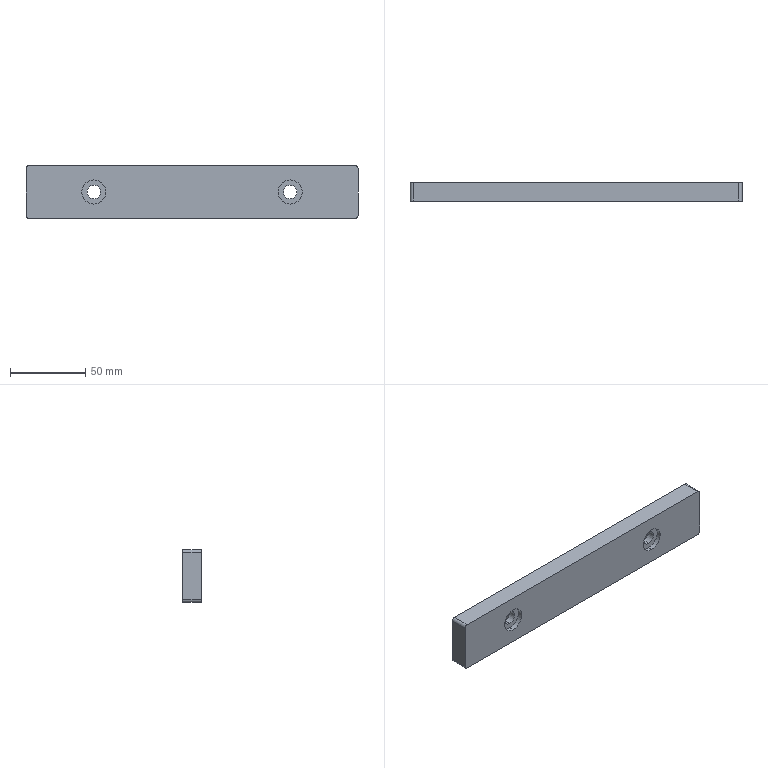Component | SolidWorks | 20-MaterialTrayLifting-1111-1_24-1111-3 | 1 solid | 24 faces | box 220 x 12 x 35 mm | volume 89259 mm3 | cylinder 12 | plane 8 | cone 4 | commonest cylinder face diameters 16 x4 9 x4 4 x4 | material A6061
build123d program:
from build123d import *

# Parameters (mm, degrees)
SKETCH1_W                                            = 220
SKETCH1_H                                            = 12
BOSS_EXTRUDE1_DEPTH                                  = 35
CONICAL_COUNTERSUNK_HOLE_FOR_M8_HEX_SOCK_D           = 9
CONICAL_COUNTERSUNK_HOLE_FOR_M8_HEX_SOCK_CSINK_D     = 17.92
CONICAL_COUNTERSUNK_HOLE_FOR_M8_HEX_SOCK_CSINK_ANGLE = 90
SKETCH5_R                                            = 8
CUT_EXTRUDE1_DEPTH                                   = 3
FILLET1_R                                            = 2


with BuildPart() as part:
    # Sketch1 → Boss-Extrude1 (new body)
    with BuildSketch(Plane.XY):
        Rectangle(SKETCH1_W, SKETCH1_H)
    extrude(amount=BOSS_EXTRUDE1_DEPTH)

    # Conical Countersunk Hole for M8 Hex Sock (through all)
    with Locations(Plane(origin=(0, 6, 0), x_dir=(1, 0, 0), z_dir=(0, 1, 0))):
        with Locations((65, -17.5), (-65, -17.5)):
            CounterSinkHole(CONICAL_COUNTERSUNK_HOLE_FOR_M8_HEX_SOCK_D / 2, CONICAL_COUNTERSUNK_HOLE_FOR_M8_HEX_SOCK_CSINK_D / 2, counter_sink_angle=CONICAL_COUNTERSUNK_HOLE_FOR_M8_HEX_SOCK_CSINK_ANGLE)

    # Sketch5 → Cut-Extrude1 (cut)
    with BuildSketch(Plane.XZ.offset(6)):
        with Locations(Location((65, 17.5, 0), (0, 0, 270))):
            Circle(SKETCH5_R)
        with Locations(Location((-65, 17.5, 0), (0, 0, 270))):
            Circle(SKETCH5_R)
    extrude(amount=-CUT_EXTRUDE1_DEPTH, mode=Mode.SUBTRACT)

    # Fillet1
    fillet1_edges = [part.edges().sort_by_distance(p)[0] for p in [
        (-110, 0, 35),
        (110, 0, 35),
        (-110, 0, 0),
        (110, 0, 0),
    ]]
    fillet(fillet1_edges, radius=FILLET1_R)


solid = part.part

# Placed as in the assembly
solid = solid.moved(Location((3.428, 542.224, 1420.556), (0, 0, 0)))
STEP:
#1=COLOUR_RGB('',0.7922,0.8196,0.9333);
#2=FILL_AREA_STYLE_COLOUR('',#1);
#3=FILL_AREA_STYLE('',(#2));
#4=SURFACE_STYLE_FILL_AREA(#3);
#5=SURFACE_SIDE_STYLE('',(#4));
#6=SURFACE_STYLE_USAGE(.BOTH.,#5);
#7=PRESENTATION_STYLE_ASSIGNMENT((#6));
#8=CARTESIAN_POINT('',(-2.424,21.229,56.931));
#9=VERTEX_POINT('',#8);
#10=CARTESIAN_POINT('',(-2.424,21.229,56.301));
#11=VERTEX_POINT('',#10);
#12=CARTESIAN_POINT('',(-2.424,21.229,56.616));
#13=DIRECTION('',(0.,-1.,0.));
#14=DIRECTION('',(0.,0.,-1.));
#15=AXIS2_PLACEMENT_3D('',#12,#13,#14);
#16=CIRCLE('',#15,0.315);
#17=EDGE_CURVE('',#9,#11,#16,.T.);
#18=ORIENTED_EDGE('',*,*,#17,.F.);
#19=CARTESIAN_POINT('',(-2.424,21.111,56.931));
#20=VERTEX_POINT('',#19);
#21=CARTESIAN_POINT('',(-2.424,21.229,56.931));
#22=DIRECTION('',(0.,-1.,0.));
#23=VECTOR('',#22,39.37);
#24=LINE('',#21,#23);
#25=EDGE_CURVE('',#9,#20,#24,.T.);
#26=ORIENTED_EDGE('',*,*,#25,.T.);
#27=CARTESIAN_POINT('',(-2.424,21.111,56.301));
#28=VERTEX_POINT('',#27);
#29=CARTESIAN_POINT('',(-2.424,21.111,56.616));
#30=DIRECTION('',(0.,-1.,0.));
#31=DIRECTION('',(0.,0.,-1.));
#32=AXIS2_PLACEMENT_3D('',#29,#30,#31);
#33=CIRCLE('',#32,0.315);
#34=EDGE_CURVE('',#20,#28,#33,.T.);
#35=ORIENTED_EDGE('',*,*,#34,.T.);
#36=CARTESIAN_POINT('',(-2.424,21.229,56.301));
#37=DIRECTION('',(0.,-1.,0.));
#38=VECTOR('',#37,39.37);
#39=LINE('',#36,#38);
#40=EDGE_CURVE('',#11,#28,#39,.T.);
#41=ORIENTED_EDGE('',*,*,#40,.F.);
#42=EDGE_LOOP('',(#18,#26,#35,#41));
#43=FACE_OUTER_BOUND('',#42,.T.);
#44=CARTESIAN_POINT('',(-2.424,21.229,56.616));
#45=DIRECTION('',(0.,-1.,0.));
#46=DIRECTION('',(0.,0.,-1.));
#47=AXIS2_PLACEMENT_3D('',#44,#45,#46);
#48=CYLINDRICAL_SURFACE('',#47,0.315);
#49=ADVANCED_FACE('',(#43),#48,.F.);
#50=CARTESIAN_POINT('',(2.694,21.229,56.931));
#51=VERTEX_POINT('',#50);
#52=CARTESIAN_POINT('',(2.694,21.229,56.301));
#53=VERTEX_POINT('',#52);
#54=CARTESIAN_POINT('',(2.694,21.229,56.616));
#55=DIRECTION('',(0.,-1.,0.));
#56=DIRECTION('',(0.,0.,-1.));
#57=AXIS2_PLACEMENT_3D('',#54,#55,#56);
#58=CIRCLE('',#57,0.315);
#59=EDGE_CURVE('',#51,#53,#58,.T.);
#60=ORIENTED_EDGE('',*,*,#59,.F.);
#61=CARTESIAN_POINT('',(2.694,21.111,56.931));
#62=VERTEX_POINT('',#61);
#63=CARTESIAN_POINT('',(2.694,21.229,56.931));
#64=DIRECTION('',(0.,-1.,0.));
#65=VECTOR('',#64,39.37);
#66=LINE('',#63,#65);
#67=EDGE_CURVE('',#51,#62,#66,.T.);
#68=ORIENTED_EDGE('',*,*,#67,.T.);
#69=CARTESIAN_POINT('',(2.694,21.111,56.301));
#70=VERTEX_POINT('',#69);
#71=CARTESIAN_POINT('',(2.694,21.111,56.616));
#72=DIRECTION('',(0.,-1.,0.));
#73=DIRECTION('',(0.,0.,-1.));
#74=AXIS2_PLACEMENT_3D('',#71,#72,#73);
#75=CIRCLE('',#74,0.315);
#76=EDGE_CURVE('',#62,#70,#75,.T.);
#77=ORIENTED_EDGE('',*,*,#76,.T.);
#78=CARTESIAN_POINT('',(2.694,21.229,56.301));
#79=DIRECTION('',(0.,-1.,0.));
#80=VECTOR('',#79,39.37);
#81=LINE('',#78,#80);
#82=EDGE_CURVE('',#53,#70,#81,.T.);
#83=ORIENTED_EDGE('',*,*,#82,.F.);
#84=EDGE_LOOP('',(#60,#68,#77,#83));
#85=FACE_OUTER_BOUND('',#84,.T.);
#86=CARTESIAN_POINT('',(2.694,21.229,56.616));
#87=DIRECTION('',(0.,-1.,0.));
#88=DIRECTION('',(0.,0.,-1.));
#89=AXIS2_PLACEMENT_3D('',#86,#87,#88);
#90=CYLINDRICAL_SURFACE('',#89,0.315);
#91=ADVANCED_FACE('',(#85),#90,.F.);
#92=CARTESIAN_POINT('',(2.694,21.408,56.439));
#93=VERTEX_POINT('',#92);
#94=CARTESIAN_POINT('',(2.694,21.408,56.794));
#95=VERTEX_POINT('',#94);
#96=CARTESIAN_POINT('',(2.694,21.408,56.616));
#97=DIRECTION('',(0.,1.,0.));
#98=DIRECTION('',(0.,0.,1.));
#99=AXIS2_PLACEMENT_3D('',#96,#97,#98);
#100=CIRCLE('',#99,0.1772);
#101=EDGE_CURVE('',#93,#95,#100,.T.);
#102=ORIENTED_EDGE('',*,*,#101,.F.);
#103=CARTESIAN_POINT('',(2.694,21.584,56.264));
#104=VERTEX_POINT('',#103);
#105=CARTESIAN_POINT('',(2.694,21.584,56.264));
#106=DIRECTION('',(0.,0.7071,-0.7071));
#107=VECTOR('',#106,39.37);
#108=LINE('',#105,#107);
#109=EDGE_CURVE('',#93,#104,#108,.T.);
#110=ORIENTED_EDGE('',*,*,#109,.T.);
#111=CARTESIAN_POINT('',(2.694,21.584,56.969));
#112=VERTEX_POINT('',#111);
#113=CARTESIAN_POINT('',(2.694,21.584,56.616));
#114=DIRECTION('',(0.,1.,0.));
#115=DIRECTION('',(0.,0.,1.));
#116=AXIS2_PLACEMENT_3D('',#113,#114,#115);
#117=CIRCLE('',#116,0.3528);
#118=EDGE_CURVE('',#104,#112,#117,.T.);
#119=ORIENTED_EDGE('',*,*,#118,.T.);
#120=CARTESIAN_POINT('',(2.694,21.584,56.969));
#121=DIRECTION('',(0.,0.7071,0.7071));
#122=VECTOR('',#121,39.37);
#123=LINE('',#120,#122);
#124=EDGE_CURVE('',#95,#112,#123,.T.);
#125=ORIENTED_EDGE('',*,*,#124,.F.);
#126=EDGE_LOOP('',(#102,#110,#119,#125));
#127=FACE_OUTER_BOUND('',#126,.T.);
#128=CARTESIAN_POINT('',(2.694,21.584,56.616));
#129=DIRECTION('',(0.,1.,0.));
#130=DIRECTION('',(0.,0.,1.));
#131=AXIS2_PLACEMENT_3D('',#128,#129,#130);
#132=CONICAL_SURFACE('',#131,0.3528,0.7854);
#133=ADVANCED_FACE('',(#127),#132,.F.);
#134=CARTESIAN_POINT('',(-2.424,21.408,56.439));
#135=VERTEX_POINT('',#134);
#136=CARTESIAN_POINT('',(-2.424,21.408,56.794));
#137=VERTEX_POINT('',#136);
#138=CARTESIAN_POINT('',(-2.424,21.408,56.616));
#139=DIRECTION('',(0.,1.,0.));
#140=DIRECTION('',(0.,0.,1.));
#141=AXIS2_PLACEMENT_3D('',#138,#139,#140);
#142=CIRCLE('',#141,0.1772);
#143=EDGE_CURVE('',#135,#137,#142,.T.);
#144=ORIENTED_EDGE('',*,*,#143,.F.);
#145=CARTESIAN_POINT('',(-2.424,21.584,56.264));
#146=VERTEX_POINT('',#145);
#147=CARTESIAN_POINT('',(-2.424,21.584,56.264));
#148=DIRECTION('',(0.,0.7071,-0.7071));
#149=VECTOR('',#148,39.37);
#150=LINE('',#147,#149);
#151=EDGE_CURVE('',#135,#146,#150,.T.);
#152=ORIENTED_EDGE('',*,*,#151,.T.);
#153=CARTESIAN_POINT('',(-2.424,21.584,56.969));
#154=VERTEX_POINT('',#153);
#155=CARTESIAN_POINT('',(-2.424,21.584,56.616));
#156=DIRECTION('',(0.,1.,0.));
#157=DIRECTION('',(0.,0.,1.));
#158=AXIS2_PLACEMENT_3D('',#155,#156,#157);
#159=CIRCLE('',#158,0.3528);
#160=EDGE_CURVE('',#146,#154,#159,.T.);
#161=ORIENTED_EDGE('',*,*,#160,.T.);
#162=CARTESIAN_POINT('',(-2.424,21.584,56.969));
#163=DIRECTION('',(0.,0.7071,0.7071));
#164=VECTOR('',#163,39.37);
#165=LINE('',#162,#164);
#166=EDGE_CURVE('',#137,#154,#165,.T.);
#167=ORIENTED_EDGE('',*,*,#166,.F.);
#168=EDGE_LOOP('',(#144,#152,#161,#167));
#169=FACE_OUTER_BOUND('',#168,.T.);
#170=CARTESIAN_POINT('',(-2.424,21.584,56.616));
#171=DIRECTION('',(0.,1.,0.));
#172=DIRECTION('',(0.,0.,1.));
#173=AXIS2_PLACEMENT_3D('',#170,#171,#172);
#174=CONICAL_SURFACE('',#173,0.3528,0.7854);
#175=ADVANCED_FACE('',(#169),#174,.F.);
#176=CARTESIAN_POINT('',(2.694,21.229,56.439));
#177=VERTEX_POINT('',#176);
#178=CARTESIAN_POINT('',(2.694,21.229,56.794));
#179=VERTEX_POINT('',#178);
#180=CARTESIAN_POINT('',(2.694,21.229,56.616));
#181=DIRECTION('',(0.,1.,0.));
#182=DIRECTION('',(0.,0.,-1.));
#183=AXIS2_PLACEMENT_3D('',#180,#181,#182);
#184=CIRCLE('',#183,0.1772);
#185=EDGE_CURVE('',#177,#179,#184,.T.);
#186=ORIENTED_EDGE('',*,*,#185,.F.);
#187=CARTESIAN_POINT('',(2.694,21.584,56.439));
#188=DIRECTION('',(0.,1.,0.));
#189=VECTOR('',#188,39.37);
#190=LINE('',#187,#189);
#191=EDGE_CURVE('',#177,#93,#190,.T.);
#192=ORIENTED_EDGE('',*,*,#191,.T.);
#193=ORIENTED_EDGE('',*,*,#101,.T.);
#194=CARTESIAN_POINT('',(2.694,21.584,56.794));
#195=DIRECTION('',(0.,1.,0.));
#196=VECTOR('',#195,39.37);
#197=LINE('',#194,#196);
#198=EDGE_CURVE('',#179,#95,#197,.T.);
#199=ORIENTED_EDGE('',*,*,#198,.F.);
#200=EDGE_LOOP('',(#186,#192,#193,#199));
#201=FACE_OUTER_BOUND('',#200,.T.);
#202=CARTESIAN_POINT('',(2.694,21.584,56.616));
#203=DIRECTION('',(0.,1.,0.));
#204=DIRECTION('',(0.,0.,1.));
#205=AXIS2_PLACEMENT_3D('',#202,#203,#204);
#206=CYLINDRICAL_SURFACE('',#205,0.1772);
#207=ADVANCED_FACE('',(#201),#206,.F.);
#208=CARTESIAN_POINT('',(-2.424,21.229,56.439));
#209=VERTEX_POINT('',#208);
#210=CARTESIAN_POINT('',(-2.424,21.229,56.794));
#211=VERTEX_POINT('',#210);
#212=CARTESIAN_POINT('',(-2.424,21.229,56.616));
#213=DIRECTION('',(0.,1.,0.));
#214=DIRECTION('',(0.,0.,-1.));
#215=AXIS2_PLACEMENT_3D('',#212,#213,#214);
#216=CIRCLE('',#215,0.1772);
#217=EDGE_CURVE('',#209,#211,#216,.T.);
#218=ORIENTED_EDGE('',*,*,#217,.F.);
#219=CARTESIAN_POINT('',(-2.424,21.584,56.439));
#220=DIRECTION('',(0.,1.,0.));
#221=VECTOR('',#220,39.37);
#222=LINE('',#219,#221);
#223=EDGE_CURVE('',#209,#135,#222,.T.);
#224=ORIENTED_EDGE('',*,*,#223,.T.);
#225=ORIENTED_EDGE('',*,*,#143,.T.);
#226=CARTESIAN_POINT('',(-2.424,21.584,56.794));
#227=DIRECTION('',(0.,1.,0.));
#228=VECTOR('',#227,39.37);
#229=LINE('',#226,#228);
#230=EDGE_CURVE('',#211,#137,#229,.T.);
#231=ORIENTED_EDGE('',*,*,#230,.F.);
#232=EDGE_LOOP('',(#218,#224,#225,#231));
#233=FACE_OUTER_BOUND('',#232,.T.);
#234=CARTESIAN_POINT('',(-2.424,21.584,56.616));
#235=DIRECTION('',(0.,1.,0.));
#236=DIRECTION('',(0.,0.,1.));
#237=AXIS2_PLACEMENT_3D('',#234,#235,#236);
#238=CYLINDRICAL_SURFACE('',#237,0.1772);
#239=ADVANCED_FACE('',(#233),#238,.F.);
#240=ORIENTED_EDGE('',*,*,#223,.F.);
#241=CARTESIAN_POINT('',(-2.424,21.229,56.616));
#242=DIRECTION('',(0.,1.,0.));
#243=DIRECTION('',(0.,0.,-1.));
#244=AXIS2_PLACEMENT_3D('',#241,#242,#243);
#245=CIRCLE('',#244,0.1772);
#246=EDGE_CURVE('',#211,#209,#245,.T.);
#247=ORIENTED_EDGE('',*,*,#246,.F.);
#248=ORIENTED_EDGE('',*,*,#230,.T.);
#249=CARTESIAN_POINT('',(-2.424,21.408,56.616));
#250=DIRECTION('',(0.,1.,0.));
#251=DIRECTION('',(0.,0.,1.));
#252=AXIS2_PLACEMENT_3D('',#249,#250,#251);
#253=CIRCLE('',#252,0.1772);
#254=EDGE_CURVE('',#137,#135,#253,.T.);
#255=ORIENTED_EDGE('',*,*,#254,.T.);
#256=EDGE_LOOP('',(#240,#247,#248,#255));
#257=FACE_OUTER_BOUND('',#256,.T.);
#258=CARTESIAN_POINT('',(-2.424,21.584,56.616));
#259=DIRECTION('',(0.,1.,0.));
#260=DIRECTION('',(0.,0.,1.));
#261=AXIS2_PLACEMENT_3D('',#258,#259,#260);
#262=CYLINDRICAL_SURFACE('',#261,0.1772);
#263=ADVANCED_FACE('',(#257),#262,.F.);
#264=ORIENTED_EDGE('',*,*,#191,.F.);
#265=CARTESIAN_POINT('',(2.694,21.229,56.616));
#266=DIRECTION('',(0.,1.,0.));
#267=DIRECTION('',(0.,0.,-1.));
#268=AXIS2_PLACEMENT_3D('',#265,#266,#267);
#269=CIRCLE('',#268,0.1772);
#270=EDGE_CURVE('',#179,#177,#269,.T.);
#271=ORIENTED_EDGE('',*,*,#270,.F.);
#272=ORIENTED_EDGE('',*,*,#198,.T.);
#273=CARTESIAN_POINT('',(2.694,21.408,56.616));
#274=DIRECTION('',(0.,1.,0.));
#275=DIRECTION('',(0.,0.,1.));
#276=AXIS2_PLACEMENT_3D('',#273,#274,#275);
#277=CIRCLE('',#276,0.1772);
#278=EDGE_CURVE('',#95,#93,#277,.T.);
#279=ORIENTED_EDGE('',*,*,#278,.T.);
#280=EDGE_LOOP('',(#264,#271,#272,#279));
#281=FACE_OUTER_BOUND('',#280,.T.);
#282=CARTESIAN_POINT('',(2.694,21.584,56.616));
#283=DIRECTION('',(0.,1.,0.));
#284=DIRECTION('',(0.,0.,1.));
#285=AXIS2_PLACEMENT_3D('',#282,#283,#284);
#286=CYLINDRICAL_SURFACE('',#285,0.1772);
#287=ADVANCED_FACE('',(#281),#286,.F.);
#288=CARTESIAN_POINT('',(4.466,21.584,57.227));
#289=VERTEX_POINT('',#288);
#290=CARTESIAN_POINT('',(4.466,21.584,56.006));
#291=VERTEX_POINT('',#290);
#292=CARTESIAN_POINT('',(4.466,21.584,57.305));
#293=DIRECTION('',(0.,0.,-1.));
#294=VECTOR('',#293,39.37);
#295=LINE('',#292,#294);
#296=EDGE_CURVE('',#289,#291,#295,.T.);
#297=ORIENTED_EDGE('',*,*,#296,.F.);
#298=CARTESIAN_POINT('',(4.466,21.111,57.227));
#299=VERTEX_POINT('',#298);
#300=CARTESIAN_POINT('',(4.466,21.111,57.227));
#301=DIRECTION('',(0.,-1.,0.));
#302=VECTOR('',#301,39.37);
#303=LINE('',#300,#302);
#304=EDGE_CURVE('',#289,#299,#303,.T.);
#305=ORIENTED_EDGE('',*,*,#304,.T.);
#306=CARTESIAN_POINT('',(4.466,21.111,56.006));
#307=VERTEX_POINT('',#306);
#308=CARTESIAN_POINT('',(4.466,21.111,57.305));
#309=DIRECTION('',(0.,0.,-1.));
#310=VECTOR('',#309,39.37);
#311=LINE('',#308,#310);
#312=EDGE_CURVE('',#299,#307,#311,.T.);
#313=ORIENTED_EDGE('',*,*,#312,.T.);
#314=CARTESIAN_POINT('',(4.466,21.584,56.006));
#315=DIRECTION('',(0.,1.,0.));
#316=VECTOR('',#315,39.37);
#317=LINE('',#314,#316);
#318=EDGE_CURVE('',#307,#291,#317,.T.);
#319=ORIENTED_EDGE('',*,*,#318,.T.);
#320=EDGE_LOOP('',(#297,#305,#313,#319));
#321=FACE_OUTER_BOUND('',#320,.T.);
#322=CARTESIAN_POINT('',(4.466,21.584,57.305));
#323=DIRECTION('',(-1.,0.,0.));
#324=DIRECTION('',(0.,0.,1.));
#325=AXIS2_PLACEMENT_3D('',#322,#323,#324);
#326=PLANE('',#325);
#327=ADVANCED_FACE('',(#321),#326,.F.);
#328=CARTESIAN_POINT('',(2.694,21.584,56.616));
#329=DIRECTION('',(0.,1.,0.));
#330=DIRECTION('',(0.,0.,1.));
#331=AXIS2_PLACEMENT_3D('',#328,#329,#330);
#332=CIRCLE('',#331,0.3528);
#333=EDGE_CURVE('',#112,#104,#332,.T.);
#334=ORIENTED_EDGE('',*,*,#333,.F.);
#335=ORIENTED_EDGE('',*,*,#118,.F.);
#336=EDGE_LOOP('',(#334,#335));
#337=FACE_BOUND('',#336,.T.);
#338=CARTESIAN_POINT('',(-2.424,21.584,56.616));
#339=DIRECTION('',(0.,1.,0.));
#340=DIRECTION('',(0.,0.,1.));
#341=AXIS2_PLACEMENT_3D('',#338,#339,#340);
#342=CIRCLE('',#341,0.3528);
#343=EDGE_CURVE('',#154,#146,#342,.T.);
#344=ORIENTED_EDGE('',*,*,#343,.F.);
#345=ORIENTED_EDGE('',*,*,#160,.F.);
#346=EDGE_LOOP('',(#344,#345));
#347=FACE_BOUND('',#346,.T.);
#348=CARTESIAN_POINT('',(4.387,21.584,57.305));
#349=VERTEX_POINT('',#348);
#350=CARTESIAN_POINT('',(-4.117,21.584,57.305));
#351=VERTEX_POINT('',#350);
#352=CARTESIAN_POINT('',(-4.196,21.584,57.305));
#353=DIRECTION('',(-1.,0.,0.));
#354=VECTOR('',#353,39.37);
#355=LINE('',#352,#354);
#356=EDGE_CURVE('',#349,#351,#355,.T.);
#357=ORIENTED_EDGE('',*,*,#356,.F.);
#358=CARTESIAN_POINT('',(4.387,21.584,57.227));
#359=DIRECTION('',(0.,1.,0.));
#360=DIRECTION('',(0.,0.,-1.));
#361=AXIS2_PLACEMENT_3D('',#358,#359,#360);
#362=CIRCLE('',#361,0.07874);
#363=EDGE_CURVE('',#349,#289,#362,.T.);
#364=ORIENTED_EDGE('',*,*,#363,.T.);
#365=ORIENTED_EDGE('',*,*,#296,.T.);
#366=CARTESIAN_POINT('',(4.387,21.584,55.927));
#367=VERTEX_POINT('',#366);
#368=CARTESIAN_POINT('',(4.387,21.584,56.006));
#369=DIRECTION('',(0.,1.,0.));
#370=DIRECTION('',(0.,0.,-1.));
#371=AXIS2_PLACEMENT_3D('',#368,#369,#370);
#372=CIRCLE('',#371,0.07874);
#373=EDGE_CURVE('',#291,#367,#372,.T.);
#374=ORIENTED_EDGE('',*,*,#373,.T.);
#375=CARTESIAN_POINT('',(-4.117,21.584,55.927));
#376=VERTEX_POINT('',#375);
#377=CARTESIAN_POINT('',(-4.196,21.584,55.927));
#378=DIRECTION('',(-1.,0.,0.));
#379=VECTOR('',#378,39.37);
#380=LINE('',#377,#379);
#381=EDGE_CURVE('',#367,#376,#380,.T.);
#382=ORIENTED_EDGE('',*,*,#381,.T.);
#383=CARTESIAN_POINT('',(-4.196,21.584,56.006));
#384=VERTEX_POINT('',#383);
#385=CARTESIAN_POINT('',(-4.117,21.584,56.006));
#386=DIRECTION('',(0.,1.,0.));
#387=DIRECTION('',(0.,0.,-1.));
#388=AXIS2_PLACEMENT_3D('',#385,#386,#387);
#389=CIRCLE('',#388,0.07874);
#390=EDGE_CURVE('',#376,#384,#389,.T.);
#391=ORIENTED_EDGE('',*,*,#390,.T.);
#392=CARTESIAN_POINT('',(-4.196,21.584,57.227));
#393=VERTEX_POINT('',#392);
#394=CARTESIAN_POINT('',(-4.196,21.584,57.305));
#395=DIRECTION('',(0.,0.,-1.));
#396=VECTOR('',#395,39.37);
#397=LINE('',#394,#396);
#398=EDGE_CURVE('',#393,#384,#397,.T.);
#399=ORIENTED_EDGE('',*,*,#398,.F.);
#400=CARTESIAN_POINT('',(-4.117,21.584,57.227));
#401=DIRECTION('',(0.,1.,0.));
#402=DIRECTION('',(0.,0.,-1.));
#403=AXIS2_PLACEMENT_3D('',#400,#401,#402);
#404=CIRCLE('',#403,0.07874);
#405=EDGE_CURVE('',#393,#351,#404,.T.);
#406=ORIENTED_EDGE('',*,*,#405,.T.);
#407=EDGE_LOOP('',(#357,#364,#365,#374,#382,#391,#399,#406));
#408=FACE_OUTER_BOUND('',#407,.T.);
#409=CARTESIAN_POINT('',(-4.196,21.584,57.305));
#410=DIRECTION('',(0.,-1.,0.));
#411=DIRECTION('',(0.,0.,-1.));
#412=AXIS2_PLACEMENT_3D('',#409,#410,#411);
#413=PLANE('',#412);
#414=ADVANCED_FACE('',(#337,#347,#408),#413,.F.);
#415=CARTESIAN_POINT('',(-4.196,21.111,57.227));
#416=VERTEX_POINT('',#415);
#417=CARTESIAN_POINT('',(-4.196,21.111,56.006));
#418=VERTEX_POINT('',#417);
#419=CARTESIAN_POINT('',(-4.196,21.111,57.305));
#420=DIRECTION('',(0.,0.,-1.));
#421=VECTOR('',#420,39.37);
#422=LINE('',#419,#421);
#423=EDGE_CURVE('',#416,#418,#422,.T.);
#424=ORIENTED_EDGE('',*,*,#423,.F.);
#425=CARTESIAN_POINT('',(-4.196,21.584,57.227));
#426=DIRECTION('',(0.,1.,0.));
#427=VECTOR('',#426,39.37);
#428=LINE('',#425,#427);
#429=EDGE_CURVE('',#416,#393,#428,.T.);
#430=ORIENTED_EDGE('',*,*,#429,.T.);
#431=ORIENTED_EDGE('',*,*,#398,.T.);
#432=CARTESIAN_POINT('',(-4.196,21.584,56.006));
#433=DIRECTION('',(0.,-1.,0.));
#434=VECTOR('',#433,39.37);
#435=LINE('',#432,#434);
#436=EDGE_CURVE('',#384,#418,#435,.T.);
#437=ORIENTED_EDGE('',*,*,#436,.T.);
#438=EDGE_LOOP('',(#424,#430,#431,#437));
#439=FACE_OUTER_BOUND('',#438,.T.);
#440=CARTESIAN_POINT('',(-4.196,21.584,57.305));
#441=DIRECTION('',(1.,0.,0.));
#442=DIRECTION('',(0.,0.,-1.));
#443=AXIS2_PLACEMENT_3D('',#440,#441,#442);
#444=PLANE('',#443);
#445=ADVANCED_FACE('',(#439),#444,.F.);
#446=CARTESIAN_POINT('',(-2.424,21.111,56.616));
#447=DIRECTION('',(0.,-1.,0.));
#448=DIRECTION('',(0.,0.,-1.));
#449=AXIS2_PLACEMENT_3D('',#446,#447,#448);
#450=CIRCLE('',#449,0.315);
#451=EDGE_CURVE('',#28,#20,#450,.T.);
#452=ORIENTED_EDGE('',*,*,#451,.F.);
#453=ORIENTED_EDGE('',*,*,#34,.F.);
#454=EDGE_LOOP('',(#452,#453));
#455=FACE_BOUND('',#454,.T.);
#456=CARTESIAN_POINT('',(2.694,21.111,56.616));
#457=DIRECTION('',(0.,-1.,0.));
#458=DIRECTION('',(0.,0.,-1.));
#459=AXIS2_PLACEMENT_3D('',#456,#457,#458);
#460=CIRCLE('',#459,0.315);
#461=EDGE_CURVE('',#70,#62,#460,.T.);
#462=ORIENTED_EDGE('',*,*,#461,.F.);
#463=ORIENTED_EDGE('',*,*,#76,.F.);
#464=EDGE_LOOP('',(#462,#463));
#465=FACE_BOUND('',#464,.T.);
#466=ORIENTED_EDGE('',*,*,#312,.F.);
#467=CARTESIAN_POINT('',(4.387,21.111,57.305));
#468=VERTEX_POINT('',#467);
#469=CARTESIAN_POINT('',(4.387,21.111,57.227));
#470=DIRECTION('',(0.,-1.,0.));
#471=DIRECTION('',(0.,0.,1.));
#472=AXIS2_PLACEMENT_3D('',#469,#470,#471);
#473=CIRCLE('',#472,0.07874);
#474=EDGE_CURVE('',#299,#468,#473,.T.);
#475=ORIENTED_EDGE('',*,*,#474,.T.);
#476=CARTESIAN_POINT('',(-4.117,21.111,57.305));
#477=VERTEX_POINT('',#476);
#478=CARTESIAN_POINT('',(-4.196,21.111,57.305));
#479=DIRECTION('',(1.,0.,0.));
#480=VECTOR('',#479,39.37);
#481=LINE('',#478,#480);
#482=EDGE_CURVE('',#477,#468,#481,.T.);
#483=ORIENTED_EDGE('',*,*,#482,.F.);
#484=CARTESIAN_POINT('',(-4.117,21.111,57.227));
#485=DIRECTION('',(0.,-1.,0.));
#486=DIRECTION('',(0.,0.,1.));
#487=AXIS2_PLACEMENT_3D('',#484,#485,#486);
#488=CIRCLE('',#487,0.07874);
#489=EDGE_CURVE('',#477,#416,#488,.T.);
#490=ORIENTED_EDGE('',*,*,#489,.T.);
#491=ORIENTED_EDGE('',*,*,#423,.T.);
#492=CARTESIAN_POINT('',(-4.117,21.111,55.927));
#493=VERTEX_POINT('',#492);
#494=CARTESIAN_POINT('',(-4.117,21.111,56.006));
#495=DIRECTION('',(0.,-1.,0.));
#496=DIRECTION('',(0.,0.,1.));
#497=AXIS2_PLACEMENT_3D('',#494,#495,#496);
#498=CIRCLE('',#497,0.07874);
#499=EDGE_CURVE('',#418,#493,#498,.T.);
#500=ORIENTED_EDGE('',*,*,#499,.T.);
#501=CARTESIAN_POINT('',(4.387,21.111,55.927));
#502=VERTEX_POINT('',#501);
#503=CARTESIAN_POINT('',(-4.196,21.111,55.927));
#504=DIRECTION('',(1.,0.,0.));
#505=VECTOR('',#504,39.37);
#506=LINE('',#503,#505);
#507=EDGE_CURVE('',#493,#502,#506,.T.);
#508=ORIENTED_EDGE('',*,*,#507,.T.);
#509=CARTESIAN_POINT('',(4.387,21.111,56.006));
#510=DIRECTION('',(0.,-1.,0.));
#511=DIRECTION('',(0.,0.,1.));
#512=AXIS2_PLACEMENT_3D('',#509,#510,#511);
#513=CIRCLE('',#512,0.07874);
#514=EDGE_CURVE('',#502,#307,#513,.T.);
#515=ORIENTED_EDGE('',*,*,#514,.T.);
#516=EDGE_LOOP('',(#466,#475,#483,#490,#491,#500,#508,#515));
#517=FACE_OUTER_BOUND('',#516,.T.);
#518=CARTESIAN_POINT('',(-4.196,21.111,57.305));
#519=DIRECTION('',(0.,1.,0.));
#520=DIRECTION('',(0.,0.,1.));
#521=AXIS2_PLACEMENT_3D('',#518,#519,#520);
#522=PLANE('',#521);
#523=ADVANCED_FACE('',(#455,#465,#517),#522,.F.);
#524=ORIENTED_EDGE('',*,*,#482,.T.);
#525=CARTESIAN_POINT('',(4.387,21.584,57.305));
#526=DIRECTION('',(0.,1.,0.));
#527=VECTOR('',#526,39.37);
#528=LINE('',#525,#527);
#529=EDGE_CURVE('',#468,#349,#528,.T.);
#530=ORIENTED_EDGE('',*,*,#529,.T.);
#531=ORIENTED_EDGE('',*,*,#356,.T.);
#532=CARTESIAN_POINT('',(-4.117,21.111,57.305));
#533=DIRECTION('',(0.,-1.,0.));
#534=VECTOR('',#533,39.37);
#535=LINE('',#532,#534);
#536=EDGE_CURVE('',#351,#477,#535,.T.);
#537=ORIENTED_EDGE('',*,*,#536,.T.);
#538=EDGE_LOOP('',(#524,#530,#531,#537));
#539=FACE_OUTER_BOUND('',#538,.T.);
#540=CARTESIAN_POINT('',(0.135,21.347,57.305));
#541=DIRECTION('',(0.,0.,1.));
#542=DIRECTION('',(1.,0.,0.));
#543=AXIS2_PLACEMENT_3D('',#540,#541,#542);
#544=PLANE('',#543);
#545=ADVANCED_FACE('',(#539),#544,.T.);
#546=ORIENTED_EDGE('',*,*,#381,.F.);
#547=CARTESIAN_POINT('',(4.387,21.347,55.927));
#548=DIRECTION('',(0.,-1.,0.));
#549=VECTOR('',#548,39.37);
#550=LINE('',#547,#549);
#551=EDGE_CURVE('',#367,#502,#550,.T.);
#552=ORIENTED_EDGE('',*,*,#551,.T.);
#553=ORIENTED_EDGE('',*,*,#507,.F.);
#554=CARTESIAN_POINT('',(-4.117,21.347,55.927));
#555=DIRECTION('',(0.,1.,0.));
#556=VECTOR('',#555,39.37);
#557=LINE('',#554,#556);
#558=EDGE_CURVE('',#493,#376,#557,.T.);
#559=ORIENTED_EDGE('',*,*,#558,.T.);
#560=EDGE_LOOP('',(#546,#552,#553,#559));
#561=FACE_OUTER_BOUND('',#560,.T.);
#562=CARTESIAN_POINT('',(0.135,21.347,55.927));
#563=DIRECTION('',(0.,0.,1.));
#564=DIRECTION('',(1.,0.,0.));
#565=AXIS2_PLACEMENT_3D('',#562,#563,#564);
#566=PLANE('',#565);
#567=ADVANCED_FACE('',(#561),#566,.F.);
#568=ORIENTED_EDGE('',*,*,#151,.F.);
#569=ORIENTED_EDGE('',*,*,#254,.F.);
#570=ORIENTED_EDGE('',*,*,#166,.T.);
#571=ORIENTED_EDGE('',*,*,#343,.T.);
#572=EDGE_LOOP('',(#568,#569,#570,#571));
#573=FACE_OUTER_BOUND('',#572,.T.);
#574=CARTESIAN_POINT('',(-2.424,21.584,56.616));
#575=DIRECTION('',(0.,1.,0.));
#576=DIRECTION('',(0.,0.,1.));
#577=AXIS2_PLACEMENT_3D('',#574,#575,#576);
#578=CONICAL_SURFACE('',#577,0.3528,0.7854);
#579=ADVANCED_FACE('',(#573),#578,.F.);
#580=ORIENTED_EDGE('',*,*,#109,.F.);
#581=ORIENTED_EDGE('',*,*,#278,.F.);
#582=ORIENTED_EDGE('',*,*,#124,.T.);
#583=ORIENTED_EDGE('',*,*,#333,.T.);
#584=EDGE_LOOP('',(#580,#581,#582,#583));
#585=FACE_OUTER_BOUND('',#584,.T.);
#586=CARTESIAN_POINT('',(2.694,21.584,56.616));
#587=DIRECTION('',(0.,1.,0.));
#588=DIRECTION('',(0.,0.,1.));
#589=AXIS2_PLACEMENT_3D('',#586,#587,#588);
#590=CONICAL_SURFACE('',#589,0.3528,0.7854);
#591=ADVANCED_FACE('',(#585),#590,.F.);
#592=CARTESIAN_POINT('',(2.694,21.229,56.616));
#593=DIRECTION('',(0.,-1.,0.));
#594=DIRECTION('',(0.,0.,-1.));
#595=AXIS2_PLACEMENT_3D('',#592,#593,#594);
#596=CIRCLE('',#595,0.315);
#597=EDGE_CURVE('',#53,#51,#596,.T.);
#598=ORIENTED_EDGE('',*,*,#597,.T.);
#599=ORIENTED_EDGE('',*,*,#59,.T.);
#600=EDGE_LOOP('',(#598,#599));
#601=FACE_OUTER_BOUND('',#600,.T.);
#602=ORIENTED_EDGE('',*,*,#270,.T.);
#603=ORIENTED_EDGE('',*,*,#185,.T.);
#604=EDGE_LOOP('',(#602,#603));
#605=FACE_BOUND('',#604,.T.);
#606=CARTESIAN_POINT('',(2.694,21.229,56.616));
#607=DIRECTION('',(0.,-1.,0.));
#608=DIRECTION('',(0.,0.,-1.));
#609=AXIS2_PLACEMENT_3D('',#606,#607,#608);
#610=PLANE('',#609);
#611=ADVANCED_FACE('',(#601,#605),#610,.T.);
#612=ORIENTED_EDGE('',*,*,#67,.F.);
#613=ORIENTED_EDGE('',*,*,#597,.F.);
#614=ORIENTED_EDGE('',*,*,#82,.T.);
#615=ORIENTED_EDGE('',*,*,#461,.T.);
#616=EDGE_LOOP('',(#612,#613,#614,#615));
#617=FACE_OUTER_BOUND('',#616,.T.);
#618=CARTESIAN_POINT('',(2.694,21.229,56.616));
#619=DIRECTION('',(0.,-1.,0.));
#620=DIRECTION('',(0.,0.,-1.));
#621=AXIS2_PLACEMENT_3D('',#618,#619,#620);
#622=CYLINDRICAL_SURFACE('',#621,0.315);
#623=ADVANCED_FACE('',(#617),#622,.F.);
#624=CARTESIAN_POINT('',(-2.424,21.229,56.616));
#625=DIRECTION('',(0.,-1.,0.));
#626=DIRECTION('',(0.,0.,-1.));
#627=AXIS2_PLACEMENT_3D('',#624,#625,#626);
#628=CIRCLE('',#627,0.315);
#629=EDGE_CURVE('',#11,#9,#628,.T.);
#630=ORIENTED_EDGE('',*,*,#629,.T.);
#631=ORIENTED_EDGE('',*,*,#17,.T.);
#632=EDGE_LOOP('',(#630,#631));
#633=FACE_OUTER_BOUND('',#632,.T.);
#634=ORIENTED_EDGE('',*,*,#246,.T.);
#635=ORIENTED_EDGE('',*,*,#217,.T.);
#636=EDGE_LOOP('',(#634,#635));
#637=FACE_BOUND('',#636,.T.);
#638=CARTESIAN_POINT('',(-2.424,21.229,56.616));
#639=DIRECTION('',(0.,-1.,0.));
#640=DIRECTION('',(0.,0.,-1.));
#641=AXIS2_PLACEMENT_3D('',#638,#639,#640);
#642=PLANE('',#641);
#643=ADVANCED_FACE('',(#633,#637),#642,.T.);
#644=ORIENTED_EDGE('',*,*,#25,.F.);
#645=ORIENTED_EDGE('',*,*,#629,.F.);
#646=ORIENTED_EDGE('',*,*,#40,.T.);
#647=ORIENTED_EDGE('',*,*,#451,.T.);
#648=EDGE_LOOP('',(#644,#645,#646,#647));
#649=FACE_OUTER_BOUND('',#648,.T.);
#650=CARTESIAN_POINT('',(-2.424,21.229,56.616));
#651=DIRECTION('',(0.,-1.,0.));
#652=DIRECTION('',(0.,0.,-1.));
#653=AXIS2_PLACEMENT_3D('',#650,#651,#652);
#654=CYLINDRICAL_SURFACE('',#653,0.315);
#655=ADVANCED_FACE('',(#649),#654,.F.);
#656=ORIENTED_EDGE('',*,*,#474,.F.);
#657=ORIENTED_EDGE('',*,*,#304,.F.);
#658=ORIENTED_EDGE('',*,*,#363,.F.);
#659=ORIENTED_EDGE('',*,*,#529,.F.);
#660=EDGE_LOOP('',(#656,#657,#658,#659));
#661=FACE_OUTER_BOUND('',#660,.T.);
#662=CARTESIAN_POINT('',(4.387,21.347,57.227));
#663=DIRECTION('',(0.,-1.,0.));
#664=DIRECTION('',(0.,0.,-1.));
#665=AXIS2_PLACEMENT_3D('',#662,#663,#664);
#666=CYLINDRICAL_SURFACE('',#665,0.07874);
#667=ADVANCED_FACE('',(#661),#666,.T.);
#668=ORIENTED_EDGE('',*,*,#514,.F.);
#669=ORIENTED_EDGE('',*,*,#551,.F.);
#670=ORIENTED_EDGE('',*,*,#373,.F.);
#671=ORIENTED_EDGE('',*,*,#318,.F.);
#672=EDGE_LOOP('',(#668,#669,#670,#671));
#673=FACE_OUTER_BOUND('',#672,.T.);
#674=CARTESIAN_POINT('',(4.387,21.584,56.006));
#675=DIRECTION('',(0.,1.,0.));
#676=DIRECTION('',(0.,0.,1.));
#677=AXIS2_PLACEMENT_3D('',#674,#675,#676);
#678=CYLINDRICAL_SURFACE('',#677,0.07874);
#679=ADVANCED_FACE('',(#673),#678,.T.);
#680=ORIENTED_EDGE('',*,*,#405,.F.);
#681=ORIENTED_EDGE('',*,*,#429,.F.);
#682=ORIENTED_EDGE('',*,*,#489,.F.);
#683=ORIENTED_EDGE('',*,*,#536,.F.);
#684=EDGE_LOOP('',(#680,#681,#682,#683));
#685=FACE_OUTER_BOUND('',#684,.T.);
#686=CARTESIAN_POINT('',(-4.117,21.347,57.227));
#687=DIRECTION('',(0.,1.,0.));
#688=DIRECTION('',(0.,0.,1.));
#689=AXIS2_PLACEMENT_3D('',#686,#687,#688);
#690=CYLINDRICAL_SURFACE('',#689,0.07874);
#691=ADVANCED_FACE('',(#685),#690,.T.);
#692=ORIENTED_EDGE('',*,*,#390,.F.);
#693=ORIENTED_EDGE('',*,*,#558,.F.);
#694=ORIENTED_EDGE('',*,*,#499,.F.);
#695=ORIENTED_EDGE('',*,*,#436,.F.);
#696=EDGE_LOOP('',(#692,#693,#694,#695));
#697=FACE_OUTER_BOUND('',#696,.T.);
#698=CARTESIAN_POINT('',(-4.117,21.584,56.006));
#699=DIRECTION('',(0.,-1.,0.));
#700=DIRECTION('',(0.,0.,-1.));
#701=AXIS2_PLACEMENT_3D('',#698,#699,#700);
#702=CYLINDRICAL_SURFACE('',#701,0.07874);
#703=ADVANCED_FACE('',(#697),#702,.T.);
#704=CLOSED_SHELL('',(#49,#91,#133,#175,#207,#239,#263,#287,#327,#414,#445,#523,#545,#567,#579,#591,#611,#623,#643,#655,#667,#679,#691,#703));
#705=MANIFOLD_SOLID_BREP('',#704);
#706=STYLED_ITEM('',(#7),#705);
#707=PRESENTATION_LAYER_ASSIGNMENT('','',(#706));
#708=CARTESIAN_POINT('',(0.,0.,0.));
#709=DIRECTION('',(0.,0.,1.));
#710=DIRECTION('',(1.,0.,0.));
#711=AXIS2_PLACEMENT_3D('',#708,#709,#710);
#712=(LENGTH_UNIT()NAMED_UNIT(*)SI_UNIT($,.METRE.));
#713=LENGTH_MEASURE_WITH_UNIT(LENGTH_MEASURE(0.0254),#712);
#714=DIMENSIONAL_EXPONENTS(1.,0.,0.,0.,0.,0.,0.);
#715=(CONVERSION_BASED_UNIT('',#713)LENGTH_UNIT()NAMED_UNIT(#714));
#716=UNCERTAINTY_MEASURE_WITH_UNIT(LENGTH_MEASURE(0.00001),#715,'','');
#717=(NAMED_UNIT(*)PLANE_ANGLE_UNIT()SI_UNIT($,.RADIAN.));
#718=(NAMED_UNIT(*)SI_UNIT($,.STERADIAN.)SOLID_ANGLE_UNIT());
#719=(GEOMETRIC_REPRESENTATION_CONTEXT(3)GLOBAL_UNCERTAINTY_ASSIGNED_CONTEXT((#716))GLOBAL_UNIT_ASSIGNED_CONTEXT((#715,#717,#718))REPRESENTATION_CONTEXT('',''));
#720=ADVANCED_BREP_SHAPE_REPRESENTATION('',(#705,#711),#719);
#721=(LENGTH_UNIT()NAMED_UNIT(*)SI_UNIT($,.METRE.));
#722=LENGTH_MEASURE_WITH_UNIT(LENGTH_MEASURE(0.0254),#721);
#723=DIMENSIONAL_EXPONENTS(1.,0.,0.,0.,0.,0.,0.);
#724=(CONVERSION_BASED_UNIT('',#722)LENGTH_UNIT()NAMED_UNIT(#723));
#725=UNCERTAINTY_MEASURE_WITH_UNIT(LENGTH_MEASURE(0.00001),#724,'','');
#726=(NAMED_UNIT(*)PLANE_ANGLE_UNIT()SI_UNIT($,.RADIAN.));
#727=(NAMED_UNIT(*)SI_UNIT($,.STERADIAN.)SOLID_ANGLE_UNIT());
#728=(GEOMETRIC_REPRESENTATION_CONTEXT(3)GLOBAL_UNCERTAINTY_ASSIGNED_CONTEXT((#725))GLOBAL_UNIT_ASSIGNED_CONTEXT((#724,#726,#727))REPRESENTATION_CONTEXT('',''));
#729=MECHANICAL_DESIGN_GEOMETRIC_PRESENTATION_REPRESENTATION('',(#706),#728);